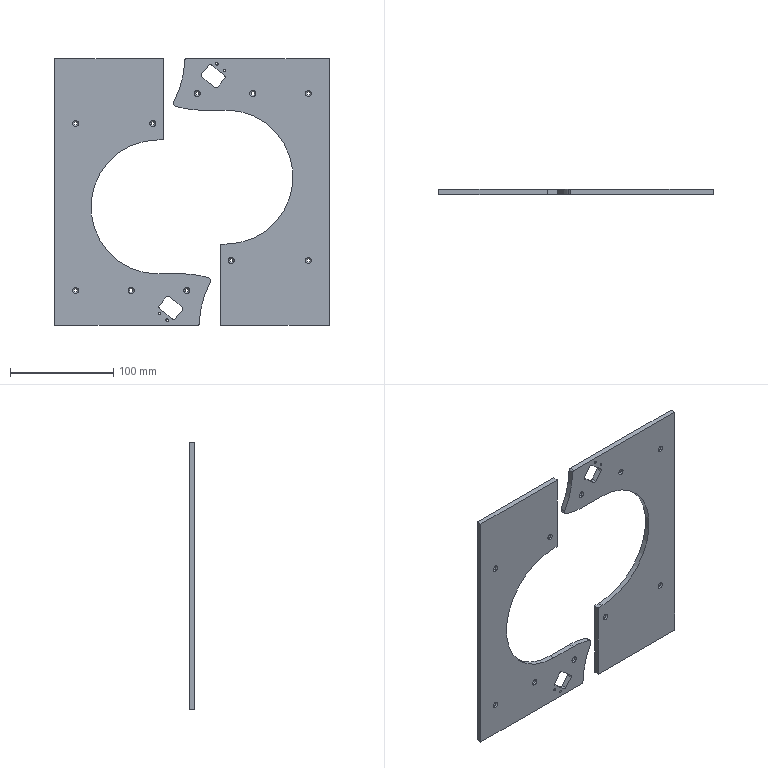CAM job | Mastercam | mm | 4 operations | part box 266 x 5 x 259
1. Contour (Ramp) | 3 - 3 平铣刀
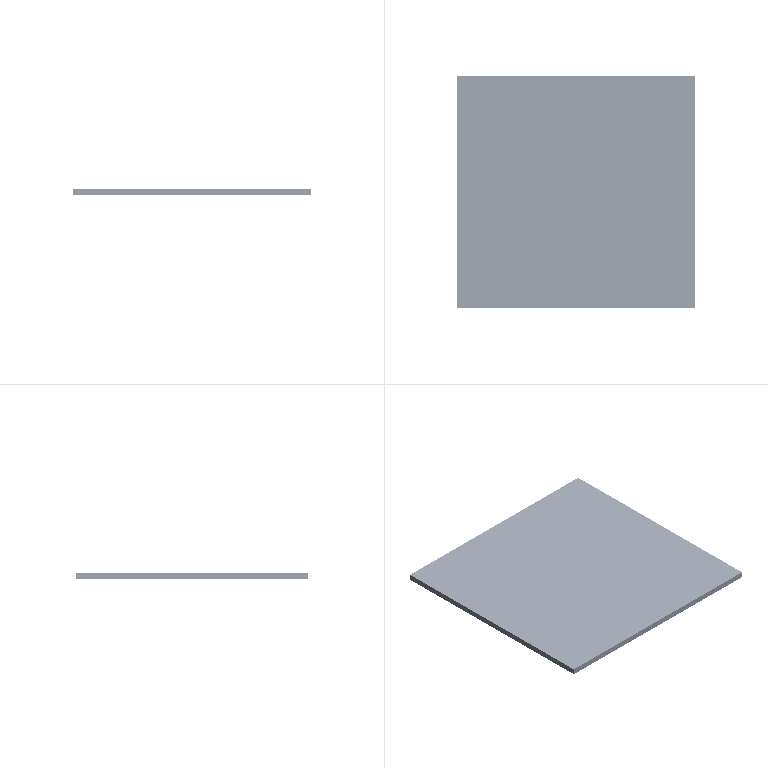2. Contour (2D) | 3 - 3 平铣刀
3. Drill/Counterbore | 7 - 4 倒角刀
4. Contour (2D chamfer) | 7 - 4 倒角刀